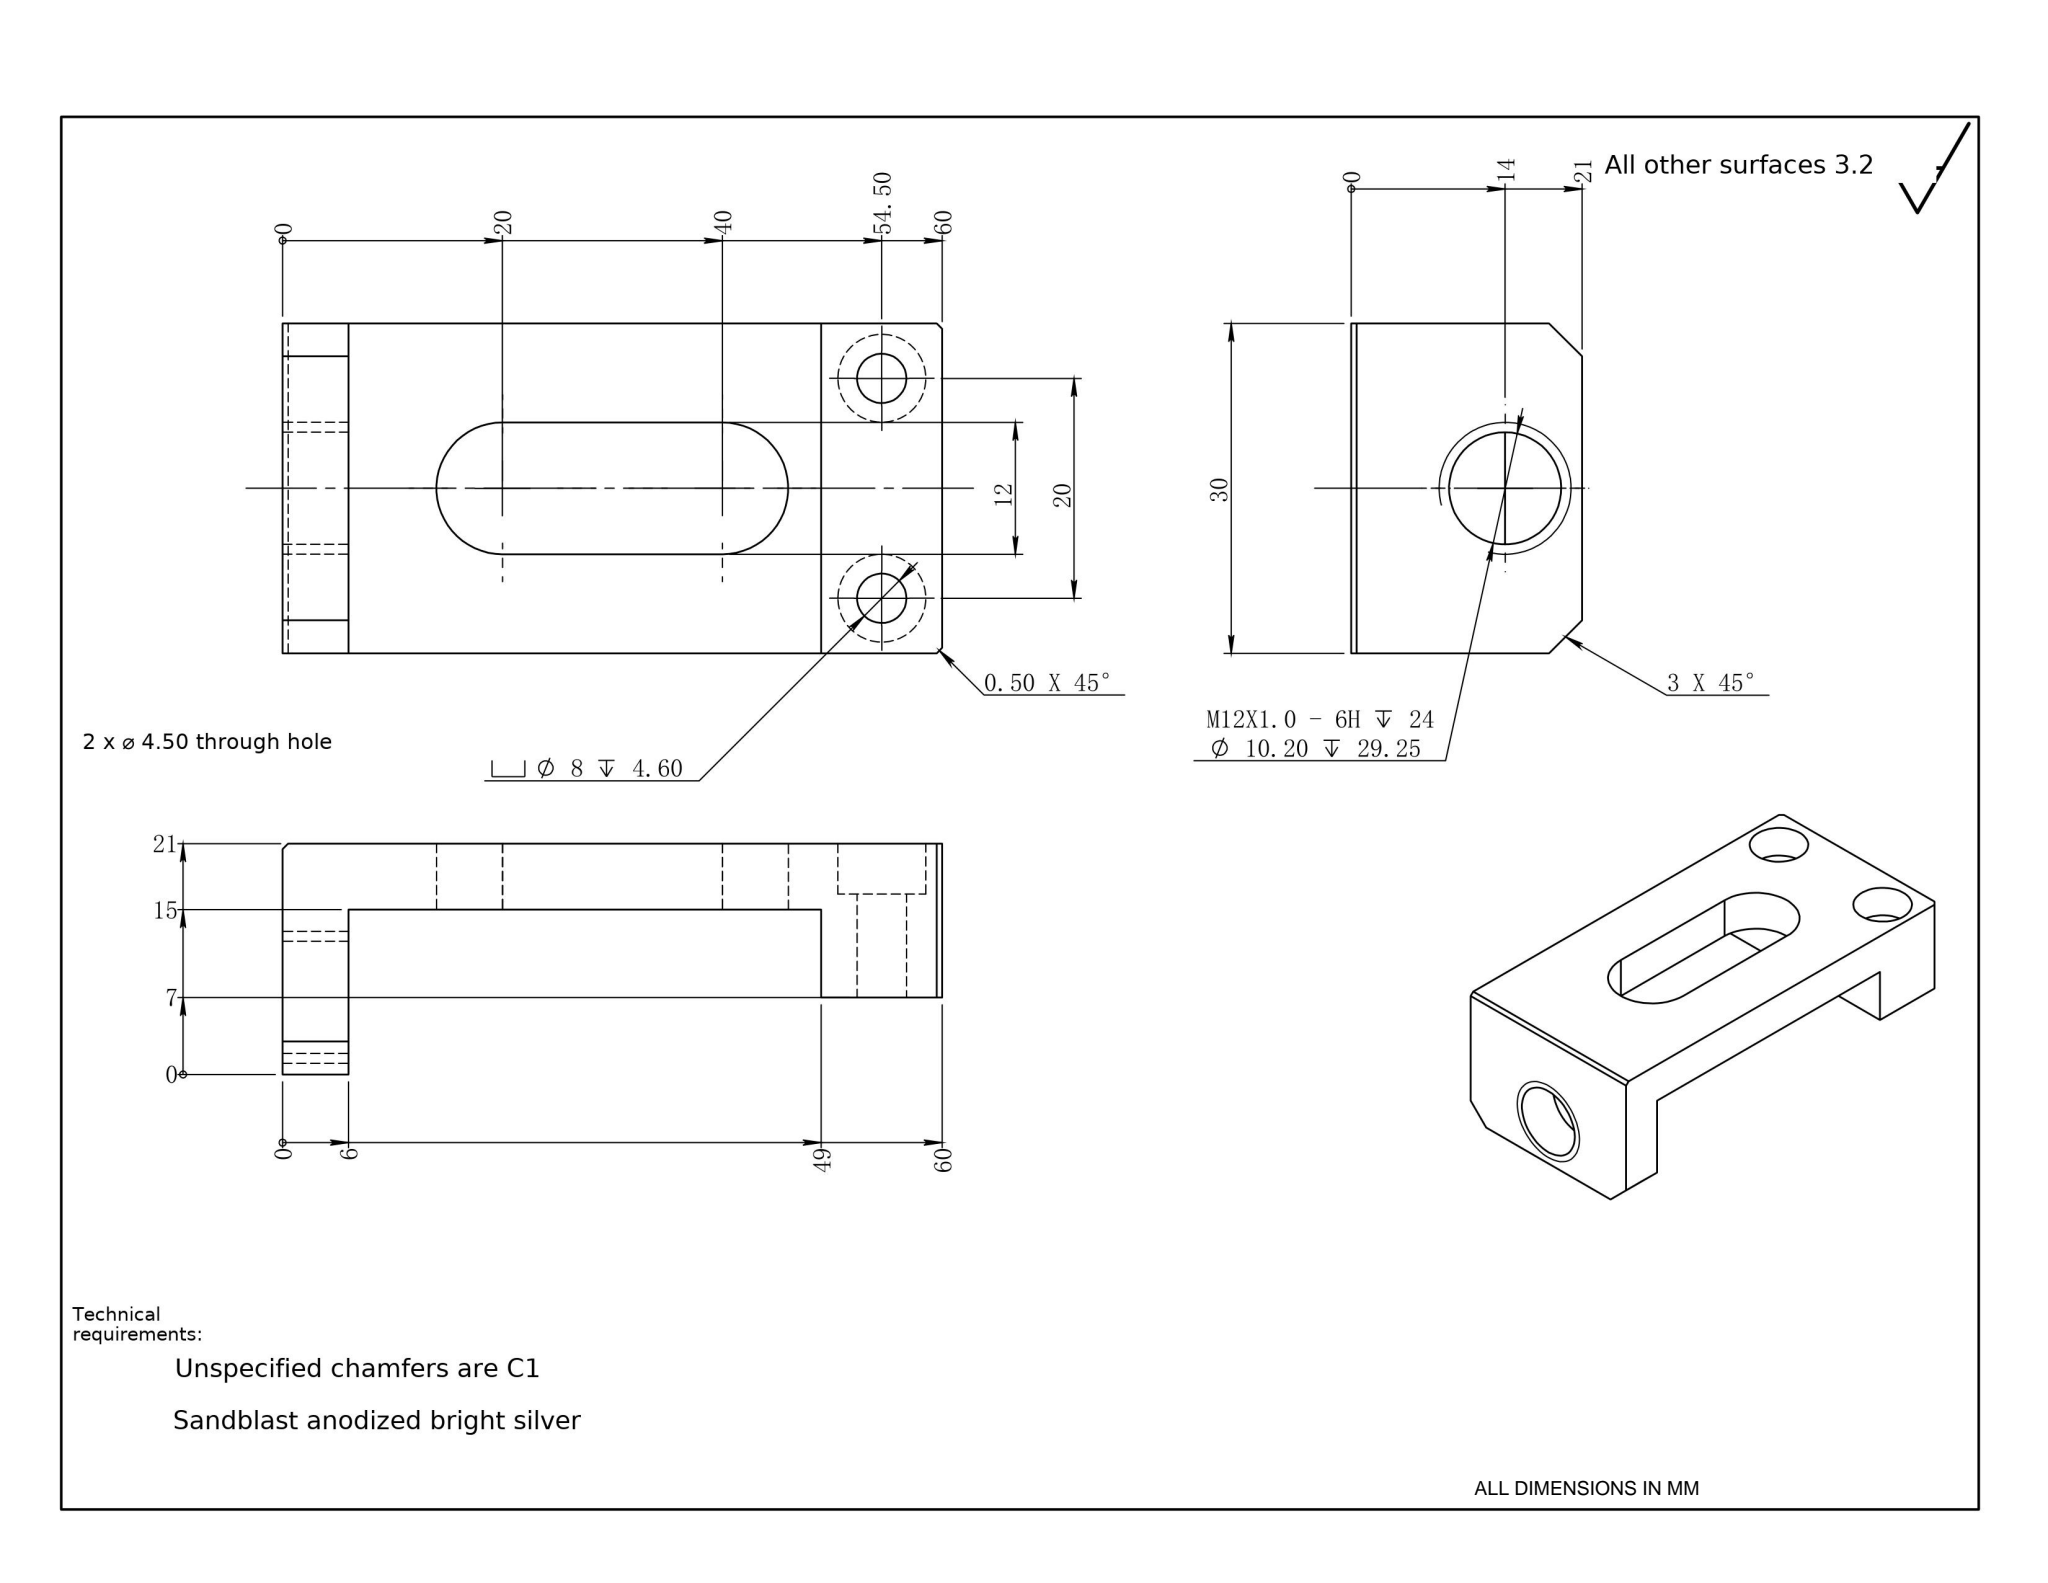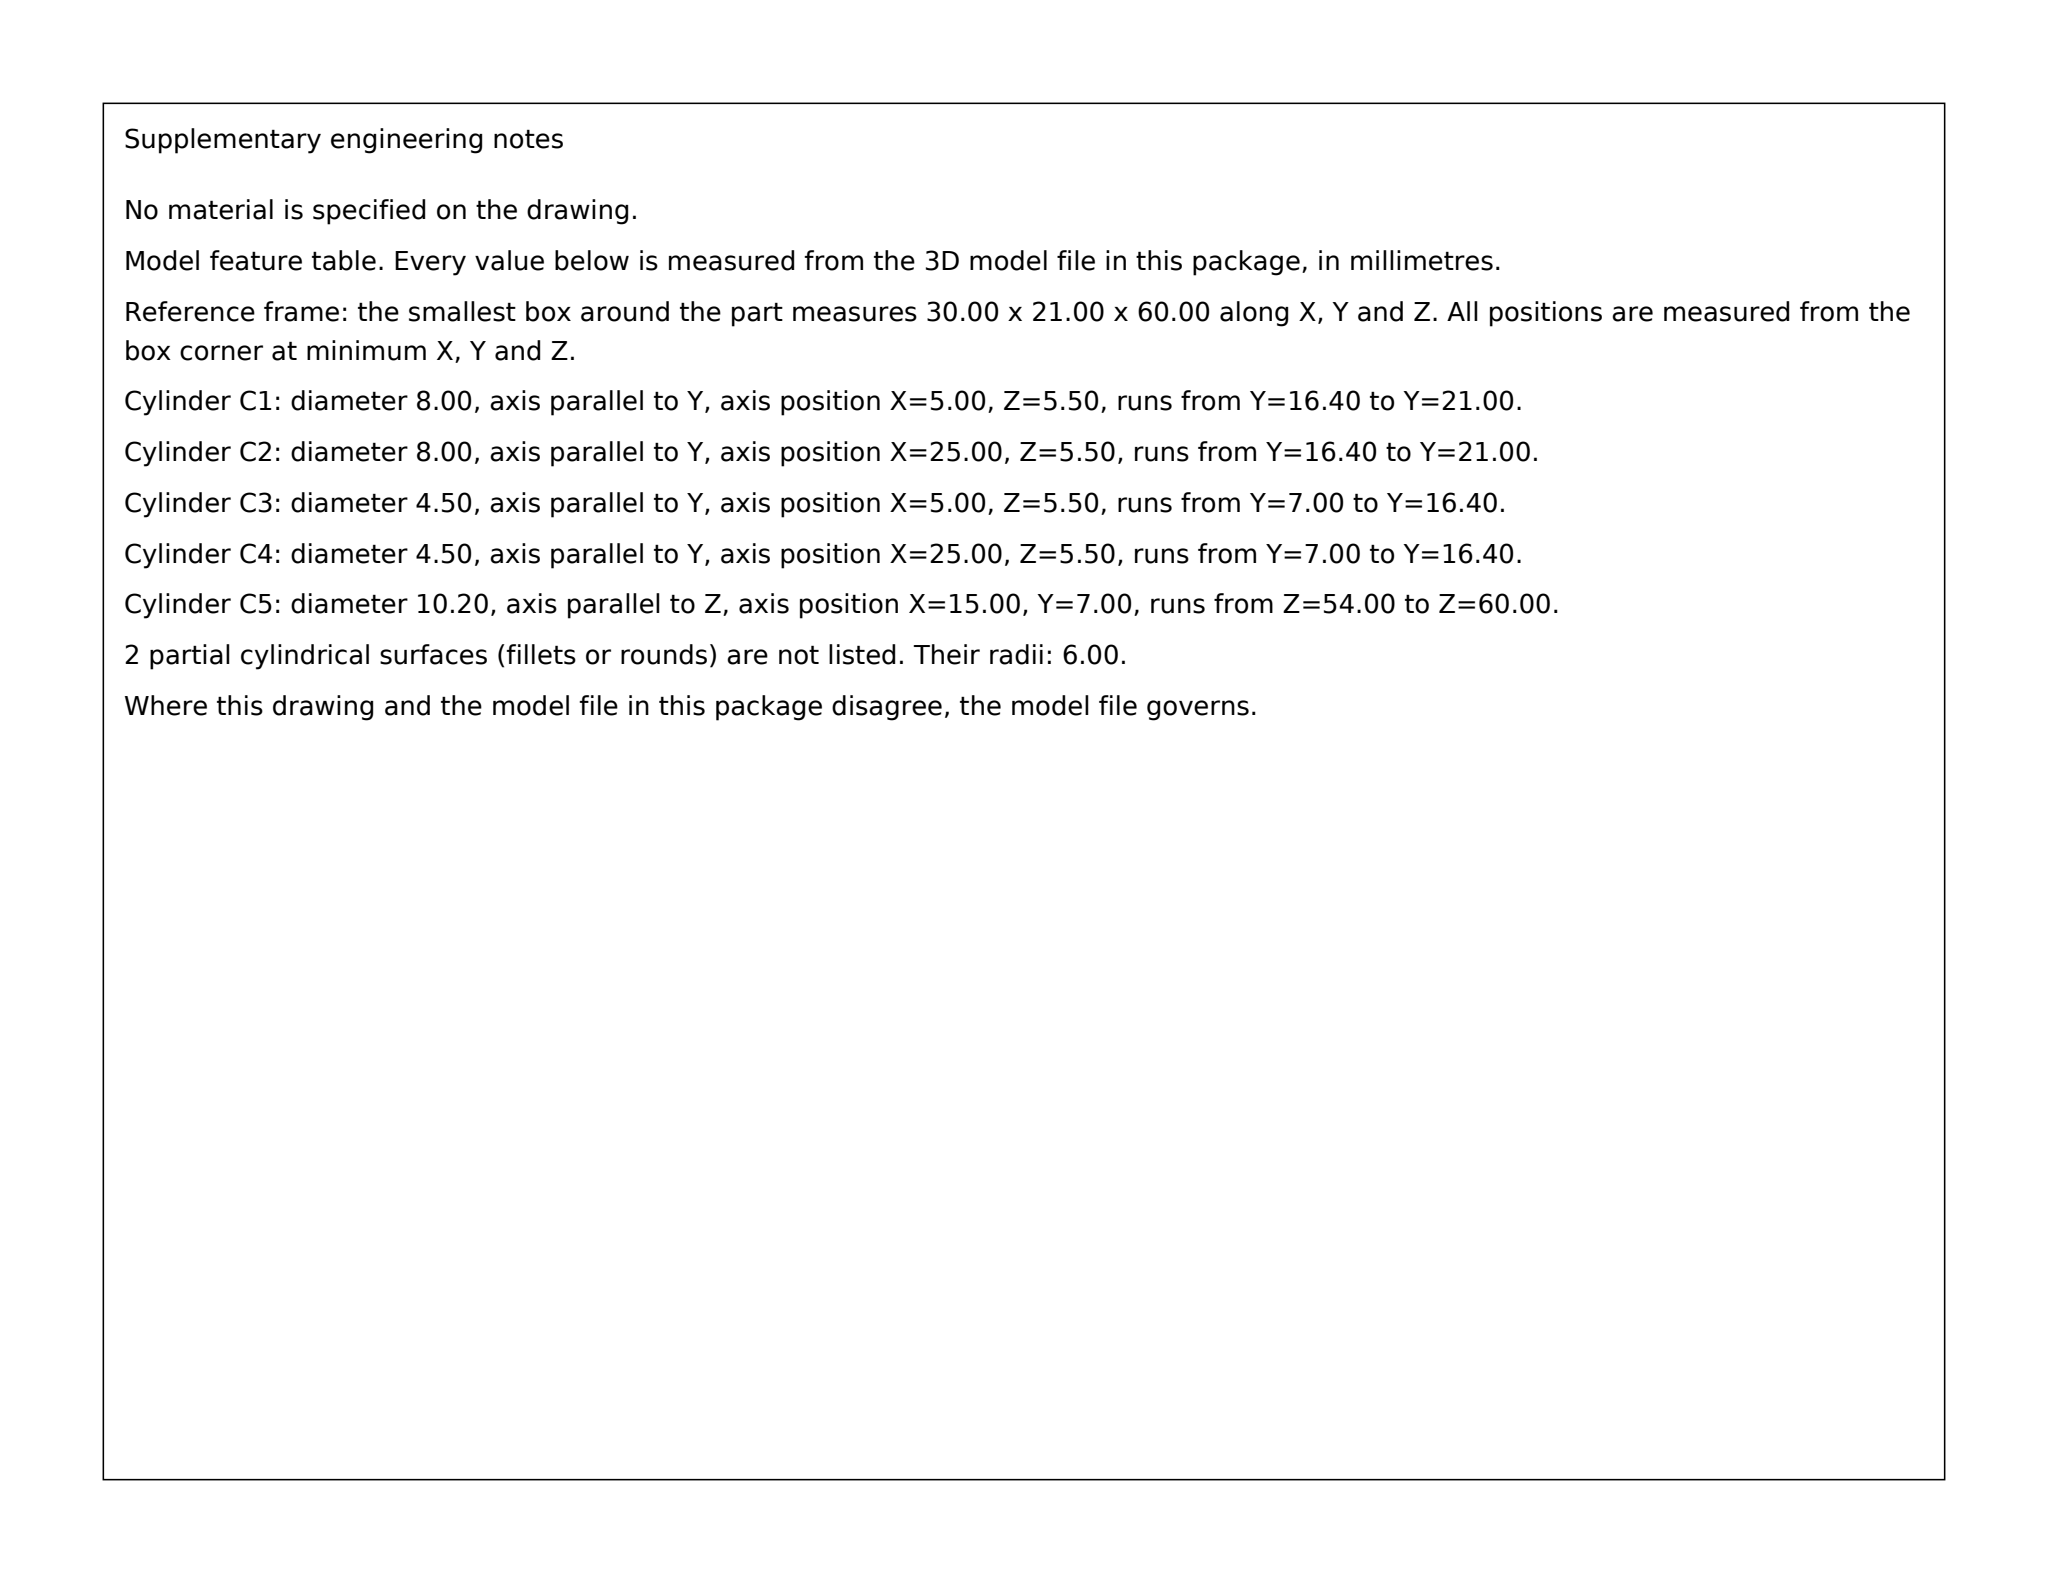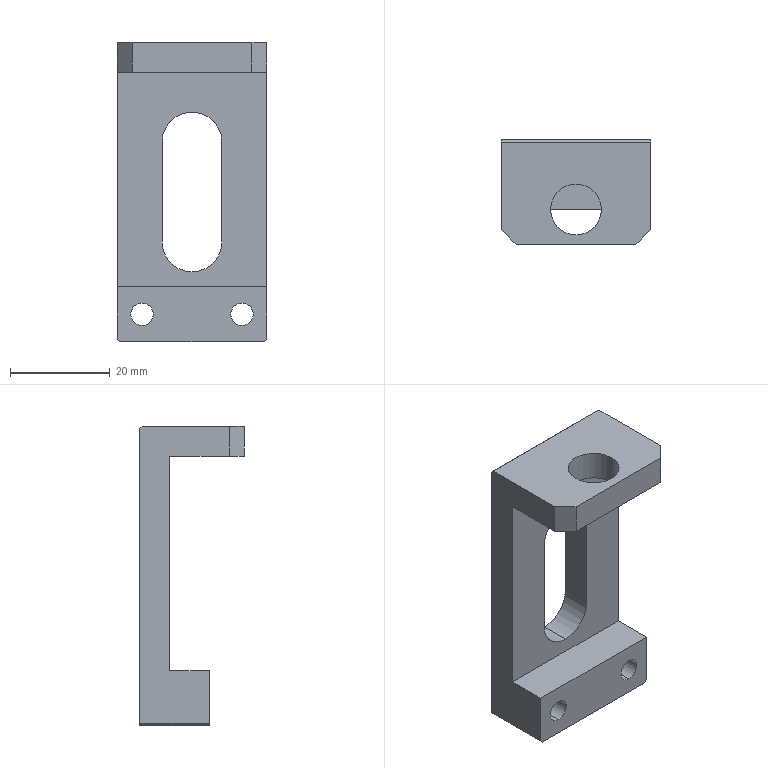Part | SolidWorks | mm | 1 solid | 32 faces | box 30 x 21 x 60 mm | volume 12708 mm3 | plane 19 | cylinder 13 | commonest cylinder face diameters 8 x4 4.5 x4 12 x3 10.2 x2
build123d program:
from build123d import *

# Parameters (mm, degrees)
SKETCH1_W                                            = 30
SKETCH1_H                                            = 6
BOSS_EXTRUDE1_DEPTH                                  = 30
SKETCH2_W                                            = 30
SKETCH2_H                                            = 11
BOSS_EXTRUDE2_DEPTH                                  = 8
SKETCH3_W                                            = 30
SKETCH3_H                                            = 6
BOSS_EXTRUDE3_DEPTH                                  = 15
CHAMFER1_SIZE                                        = 3
M12_TAPPED_HOLE1_D                                   = 10.2
M12_TAPPED_HOLE1_DEPTH                               = 29.25
M12_TAPPED_HOLE1_TIP                                 = 3.064
CUT_EXTRUDE1_DEPTH                                   = 37.742
HOLE_SIZE_ACCORDING_TO_THE_TYPE_OF_HEXAG_D           = 4.5
HOLE_SIZE_ACCORDING_TO_THE_TYPE_OF_HEXAG_CBORE_D     = 8
HOLE_SIZE_ACCORDING_TO_THE_TYPE_OF_HEXAG_CBORE_DEPTH = 4.6
CHAMFER2_SIZE                                        = 0.5


with BuildPart() as part:
    # Sketch1 → Boss-Extrude1 (new, symmetric)
    with BuildSketch(Plane.XY):
        Rectangle(SKETCH1_W, SKETCH1_H)
    extrude(amount=BOSS_EXTRUDE1_DEPTH, both=True)

    # Sketch2 → Boss-Extrude2 (add)
    with BuildSketch(Plane.XZ.offset(3)):
        with Locations((0, -24.5)):
            Rectangle(SKETCH2_W, SKETCH2_H)
    extrude(amount=BOSS_EXTRUDE2_DEPTH)

    # Sketch3 → Boss-Extrude3 (add)
    with BuildSketch(Plane.XZ.offset(3)):
        with Locations((0, 27)):
            Rectangle(SKETCH3_W, SKETCH3_H)
    extrude(amount=BOSS_EXTRUDE3_DEPTH)

    # Chamfer1
    chamfer1_edges = [part.edges().sort_by_distance(p)[0] for p in [
        (-15, -18, 27),
        (15, -18, 27),
    ]]
    chamfer(chamfer1_edges, length=CHAMFER1_SIZE)

    # M12 Tapped Hole1
    with Locations(Plane.XY.offset(30)):
        with Locations((0, -11)):
            Hole(M12_TAPPED_HOLE1_D / 2, depth=M12_TAPPED_HOLE1_DEPTH)
            with Locations((0, 0, -(M12_TAPPED_HOLE1_DEPTH + M12_TAPPED_HOLE1_TIP / 2))):  # 118° drill point
                Cone(0, M12_TAPPED_HOLE1_D / 2, M12_TAPPED_HOLE1_TIP, mode=Mode.SUBTRACT)

    # Sketch6 → Cut-Extrude1 (cut, through all)
    with BuildSketch(Plane.XZ.offset(3)):
        with BuildLine():
            Line((6, 10), (6, -10))
            ThreePointArc((6, -10), (0, -16), (-6, -10))
            Line((-6, -10), (-6, 10))
            ThreePointArc((-6, 10), (0, 16), (6, 10))
        make_face()
    extrude(amount=-CUT_EXTRUDE1_DEPTH, mode=Mode.SUBTRACT)

    # Hole size according to the type of hexag (through all)
    with Locations(Plane(origin=(0, 3, 0), x_dir=(1, 0, 0), z_dir=(0, 1, 0))):
        with Locations((-10, 24.5), (10, 24.5)):
            CounterBoreHole(HOLE_SIZE_ACCORDING_TO_THE_TYPE_OF_HEXAG_D / 2, HOLE_SIZE_ACCORDING_TO_THE_TYPE_OF_HEXAG_CBORE_D / 2, HOLE_SIZE_ACCORDING_TO_THE_TYPE_OF_HEXAG_CBORE_DEPTH)

    # Chamfer2
    chamfer2_edges = [part.edges().sort_by_distance(p)[0] for p in [
        (-15, -4, -30),
        (15, -4, -30),
        (0, 3, 30),
    ]]
    chamfer(chamfer2_edges, length=CHAMFER2_SIZE)


solid = part.part